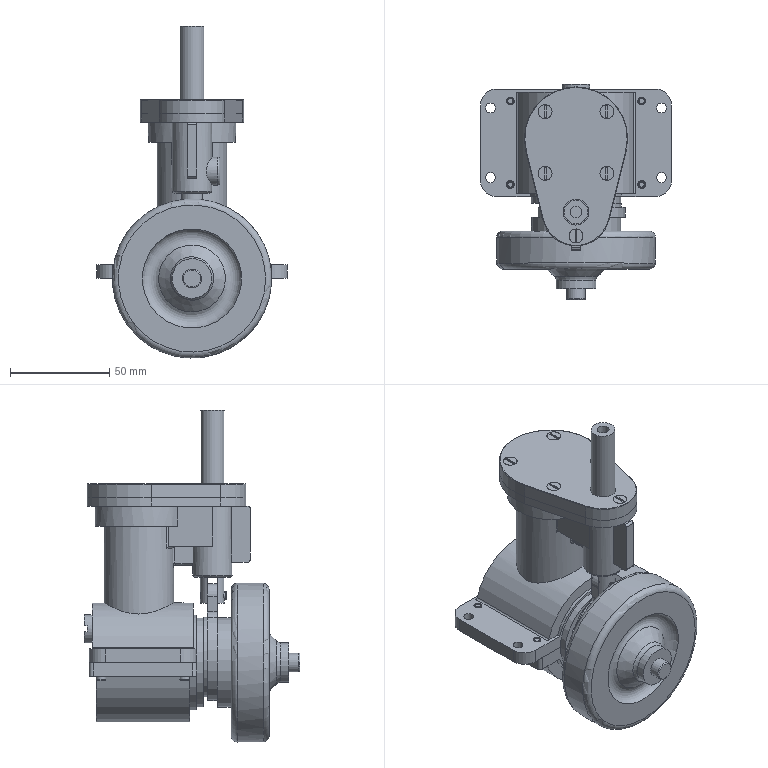Assembly | NX | mm | 27 component files | 27 solids | 402 faces | box 96 x 108.5 x 167 mm | volume 319145 mm3 | plane 195 | cylinder 139 | cone 42 | torus 24 | spline 2 | commonest cylinder face diameters 4 x30 5 x15 2 x10 12 x6 3.3 x6 7 x5 26 x4 8 x4
Bill of materials:
unnamed part 1 | 1 |  | Flanged hub: a thin circular flange with three bolt holes and a central through bore. A long plain tube sticks out on one side, and a stepped two-diameter boss sits on the other.
unnamed part 2 | 1 |  | Complex housing. A rectangular base plate with rounded corners carries a half-cylinder saddle and an upright cylindrical tower. The tower ends in a teardrop-shaped top plate with one large bore, one small bore and several small holes. There is a side boss with a hole and a flat rectangular pad on the side.
unnamed part 3 | 1 |  | Hollow stepped cylinder: a long tube with a short, smaller-diameter spigot at one end and an axial through bore.
unnamed part 4 | 1 |  | Thin, flat split ring with a rectangular cross-section and a single angled cut through the ring.
unnamed part 5 | 1 |  | Short cylinder with a flat closed top, one circumferential groove near the top, and a cross hole through the side wall.
unnamed part 6 | 1 |  | Plain cylindrical sleeve or tube, with a length roughly equal to its outer diameter and a relatively thin wall.
unnamed part 7 | 1 |  | Stepped pin. A cylindrical head joins a reduced neck, followed by a larger collar and a body. The body ends in a slotted, forked end with a cross hole.
unnamed part 8 | 1 |  | Shouldered pin: a round head with a rounded edge, a larger shank, and a smaller end shank with a chamfered tip.
unnamed part 9 | 1 |  | Half-cylinder trough or cover housing with a rectangular mounting flange, four corner holes, a rectangular opening into a curved cavity, and a semicircular cutout at one end.
unnamed part 10 | 1 |  | Plain solid cylindrical rod or pin with flat ends and small edge breaks.
unnamed part 11 | 1 |  | Plain cylindrical tube or sleeve, longer than its outer diameter, with a concentric through bore.
unnamed part 12 | 1 |  | Link or rod with a cylindrical eye at each end, joined by a tapered web with an I-section.
unnamed part 13 | 1 |  | Stepped cylindrical pin: a longer large-diameter section and a shorter, smaller-diameter coaxial section with a chamfered free end; a straight slot runs across the end face of the large-diameter section.
unnamed part 14 | 1 |  | Short flanged cylindrical spigot: a wide disc-shaped flange with a rectangular slot across its outer face, and a smaller coaxial cylindrical boss with a chamfered end on the other side.
unnamed part 15 | 5 |  | Countersunk-style slotted head on a plain cylindrical shank: a conical head with a flat top face, a straight slot across the top, and a chamfered shank end.
unnamed part 16 | 4 |  | Headed cylindrical pin: a long, slender plain cylindrical shank with a chamfered end, and a short, larger-diameter cylindrical head with a chamfered outer edge.
unnamed part 17 | 1 |  | Wheel- or roller-like rotational part: a wide disc rim with rounded edges, a recessed face, and a central hub with a small through bore. The hub stands out on both sides, conical on one side and stepped cylindrical on the other.
unnamed part 18 | 1 |  | Flat teardrop-shaped plate of constant thickness with six small countersunk or chamfered through holes near the perimeter, and one larger through hole near the narrow end with a shallow counterbore or annular groove around it on one face.
unnamed part 19 | 1 |  | Flat annular ring with a single radial tab carrying a small through hole. One face has a slightly raised or stepped region, so the part shows two thickness levels.
unnamed part 20 | 1 |  | Plate-mounted pin: an irregular, roughly tapered flat plate with a curved wide edge, a small offset through hole near the narrow rounded end, and a long plain cylindrical pin standing perpendicular from the plate face.
Mates:
1. fix | bottom_casing 1 component
2. concentric | engine_body 1 edge | bottom_casing 1 edge
3. parallel | bottom_casing 1 face | engine_body 1 face
4. concentric | top_casing 1 arc | engine_body 1 edge
5. parallel | top_casing 1 face | engine_body 1 face
6. concentric | engine_body 1 edge | flywheel_shaft 1 arc
7. concentric | bottom_casing 1 edge | flywheel_shaft 1 arc
8. concentric | breather_pipe 1 edge | top_casing 1 edge
9. concentric | bolt_M8X5 1 edge | engine_body 1 edge
10. parallel | bolt_M8X5 1 face | engine_body 1 face
11. touch align | crankshaft 1 face | flywheel 1 face
12. concentric | flywheel_shaft 1 edge | flywheel 1 arc
13. concentric | piston_ring 1 arc | piston 1 edge
14. touch align | piston_pin 1 face | piston 1 face
15. center | piston_pin 1 face | piston_pin 1 face | piston 1 face
16. touch align | connecting_rod 1 face | piston_pin 1 face
17. center | connecting_rod 1 face | connecting_rod 1 face | piston 1 face
18. concentric | top_bearing_shell 1 arc | connecting_rod 1 edge
19. concentric | bottom_bearing_shell 1 arc | connecting_rod 1 edge
20. touch align | piston 1 face | engine_body 1 face
21. concentric | bottom_bearing_shell 1 arc | crankshaft 1 edge
22. concentric | connecting_pin 1 edge | bottom_bearing_shell 1 edge
23. touch align | pin 1 face | small_piston 1 face
24. touch align | small_piston 1 face | pin 1 face
25. touch align | small_piston 1 face | engine_body 1 face
26. parallel | small_piston 1 face | swivel_ring 1 face
27. distance | pin 1 face | swivel_ring 1 face
28. distance | swivel_ring 1 face | flywheel 1 face
29. touch align | swivel_ring 1 face | small_piston 1 face
30. concentric | fixing_screw 5 edge | top_casing 1 edge
31. concentric | fixing_screw 4 edge | top_casing 1 edge
32. concentric | fixing_screw 3 edge | top_casing 1 edge
33. concentric | fixing_screw 2 edge | top_casing 1 edge
34. concentric | fixing_screw 1 edge | top_casing 1 edge
35. concentric | screw_M3X12prt 4 edge | bottom_casing 1 edge
36. concentric | screw_M3X12prt 3 edge | bottom_casing 1 edge
37. concentric | screw_M3X12prt 2 edge | bottom_casing 1 edge
38. concentric | screw_M3X12prt 1 edge | bottom_casing 1 edge